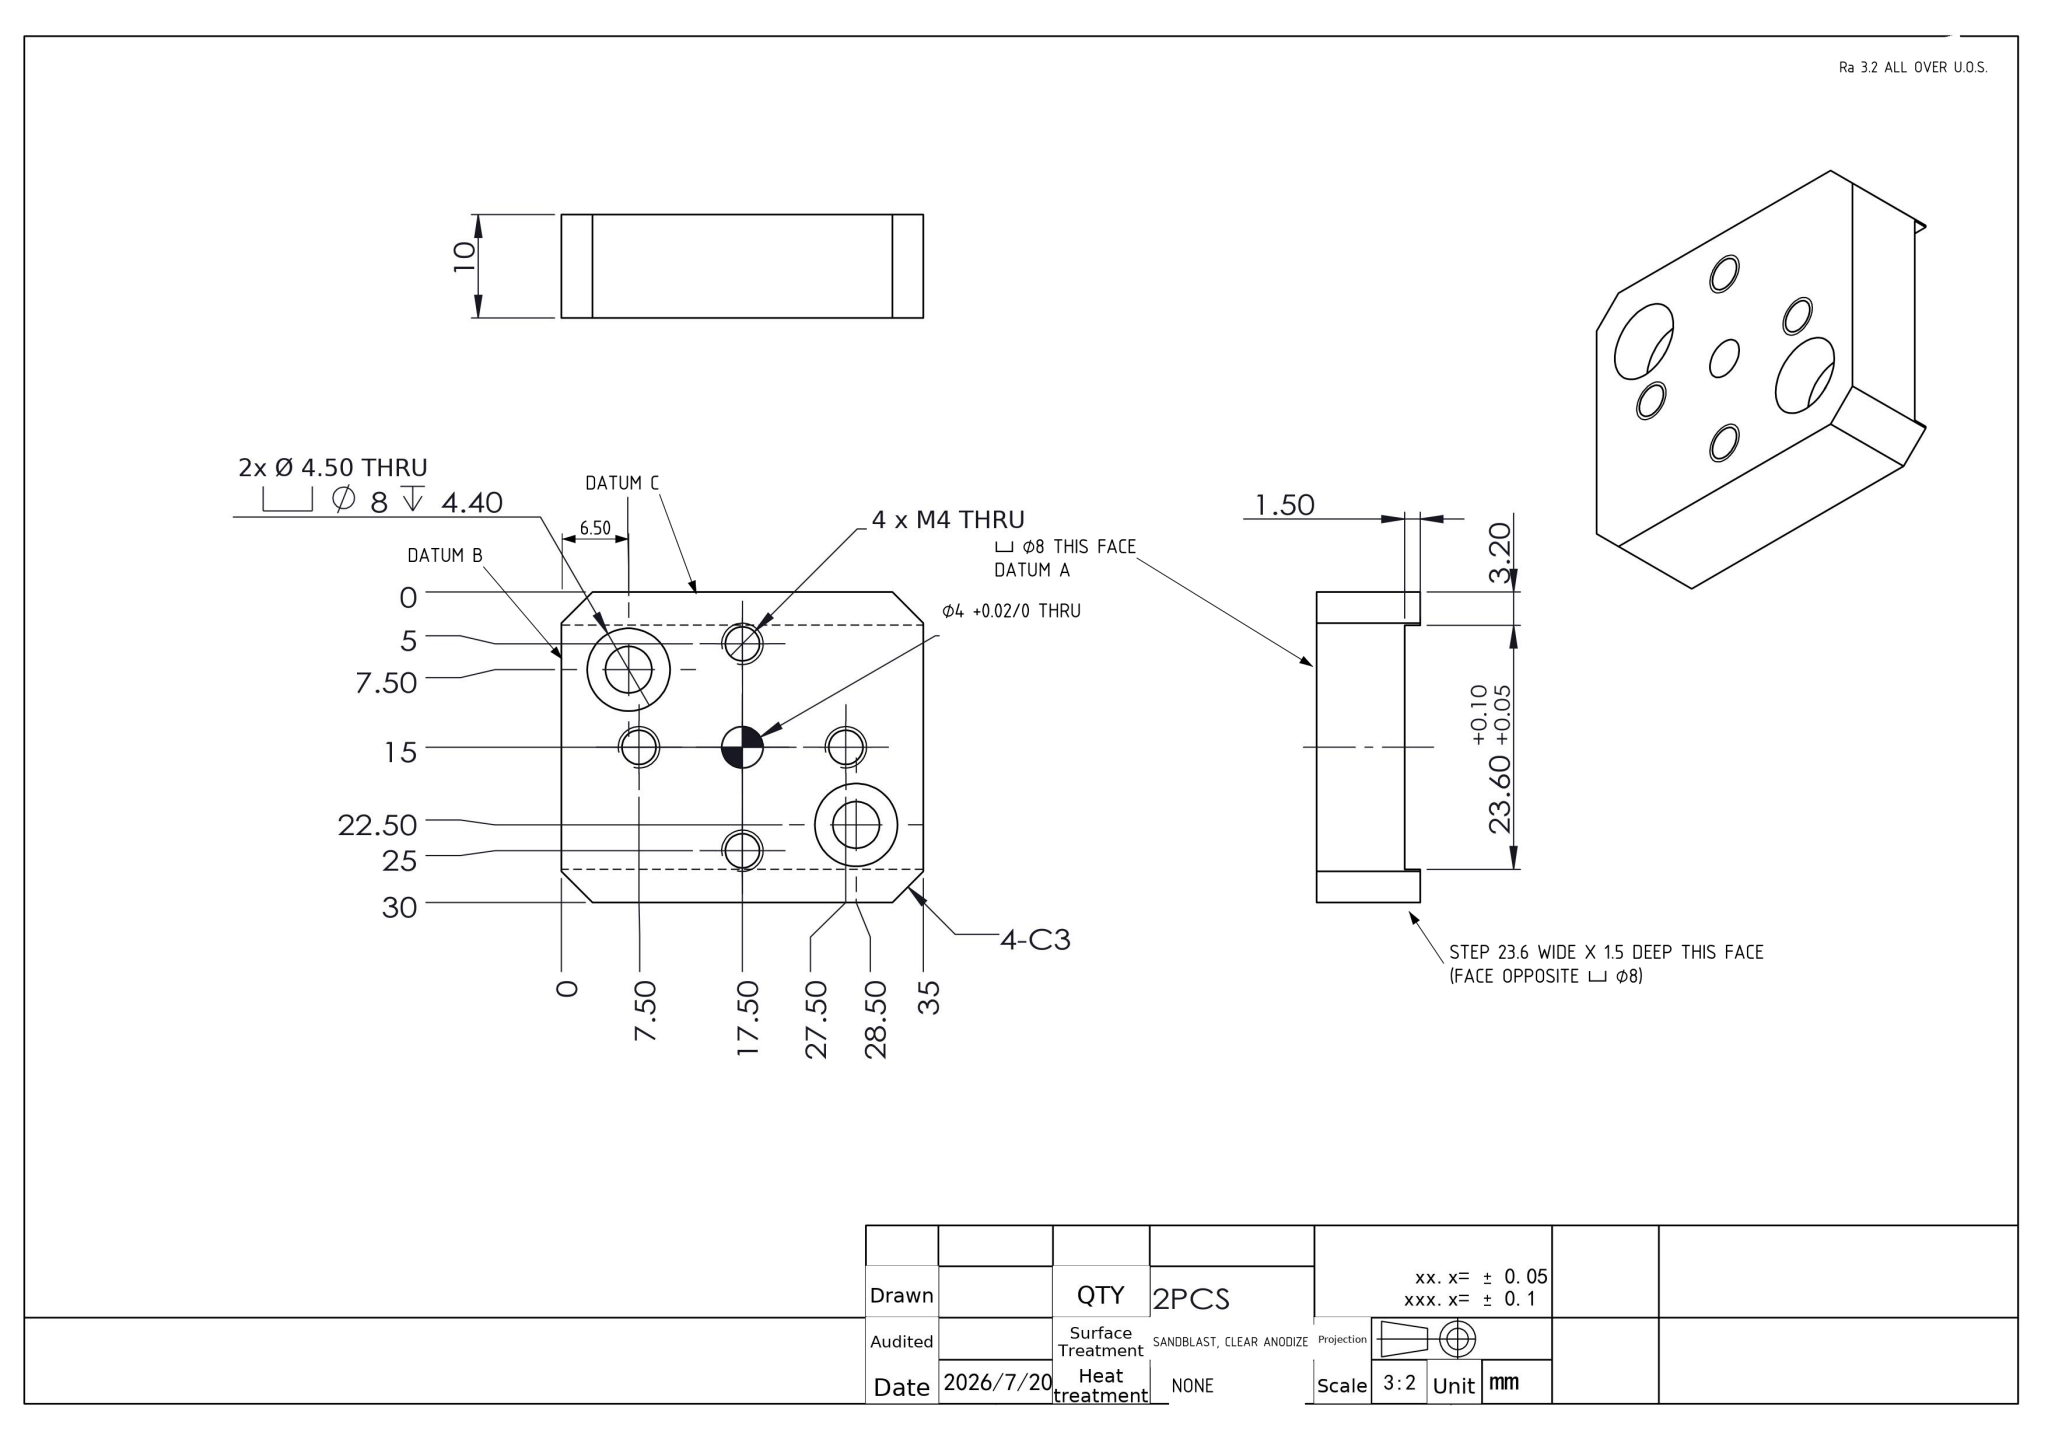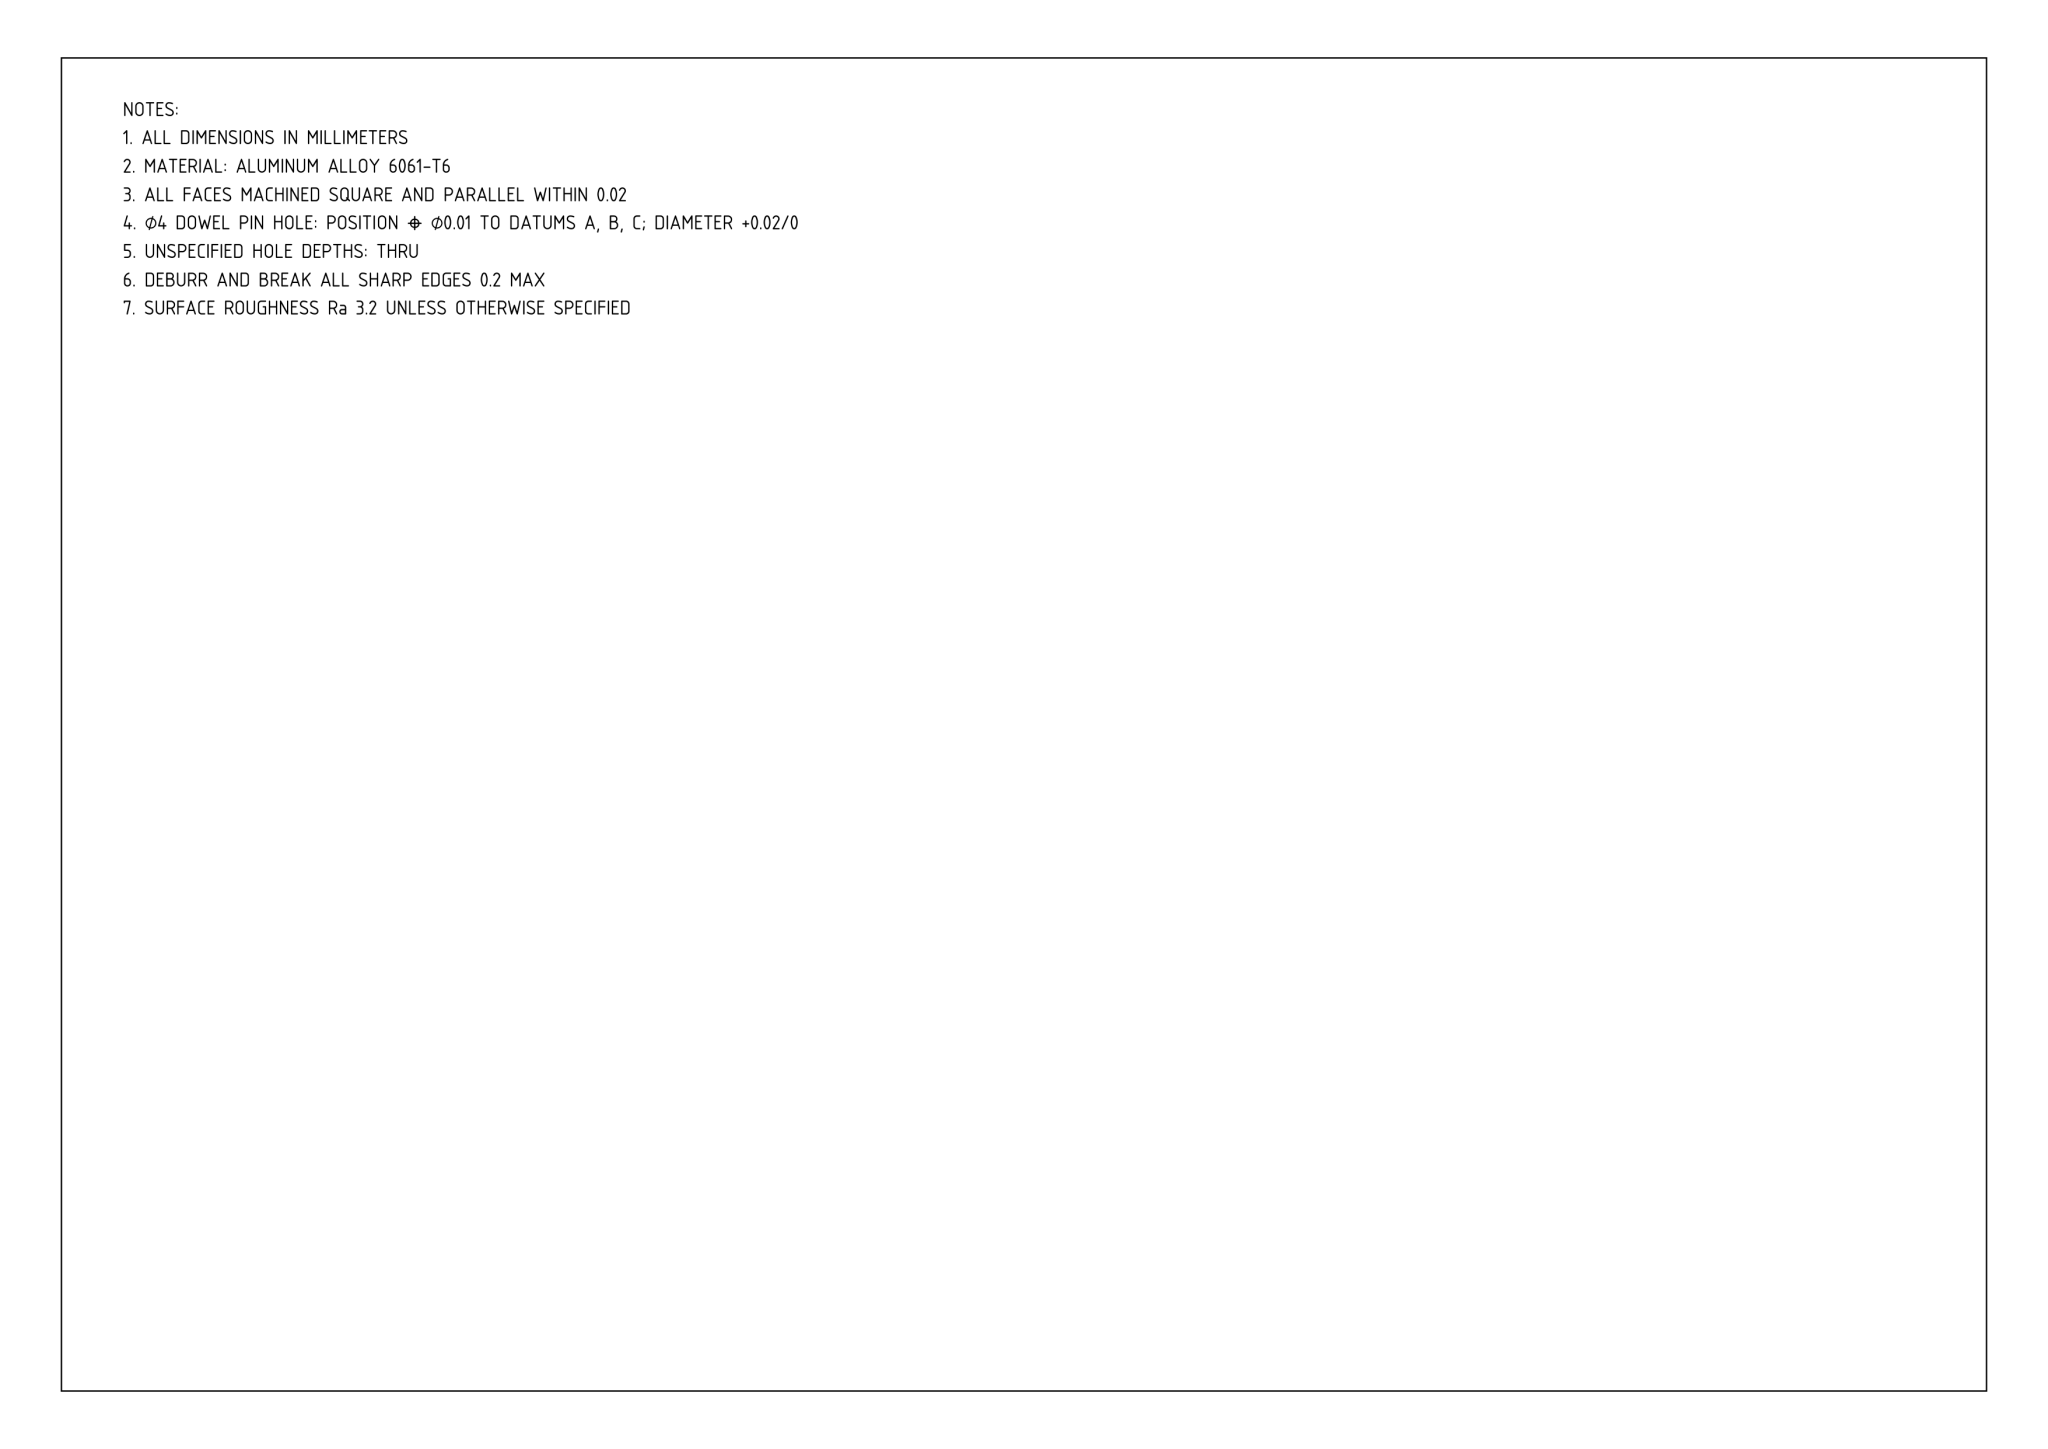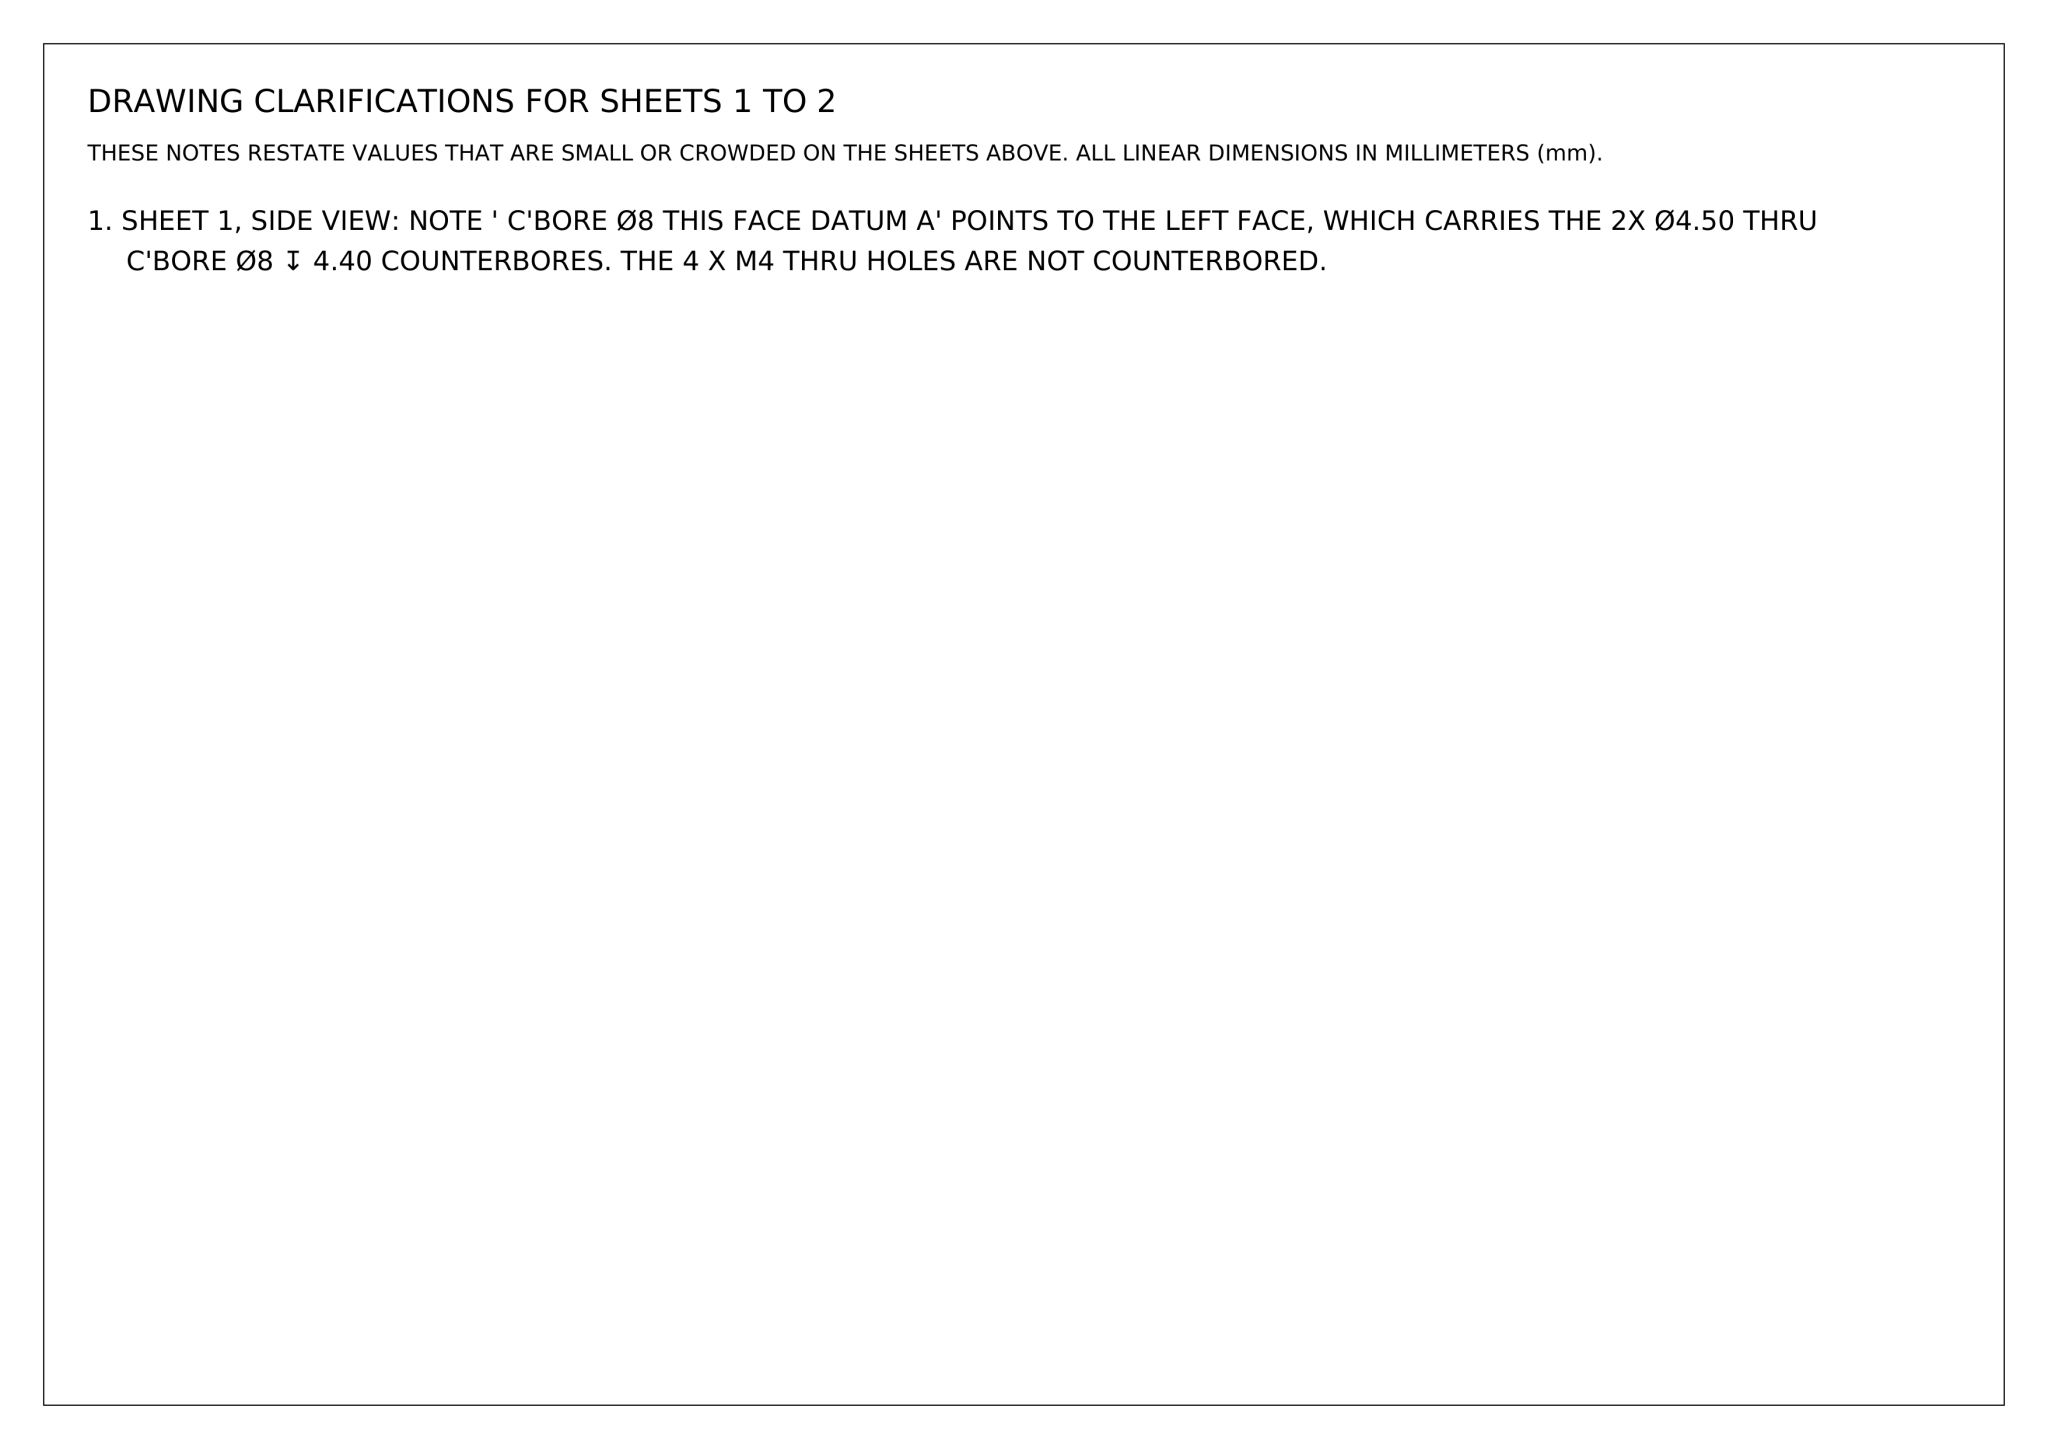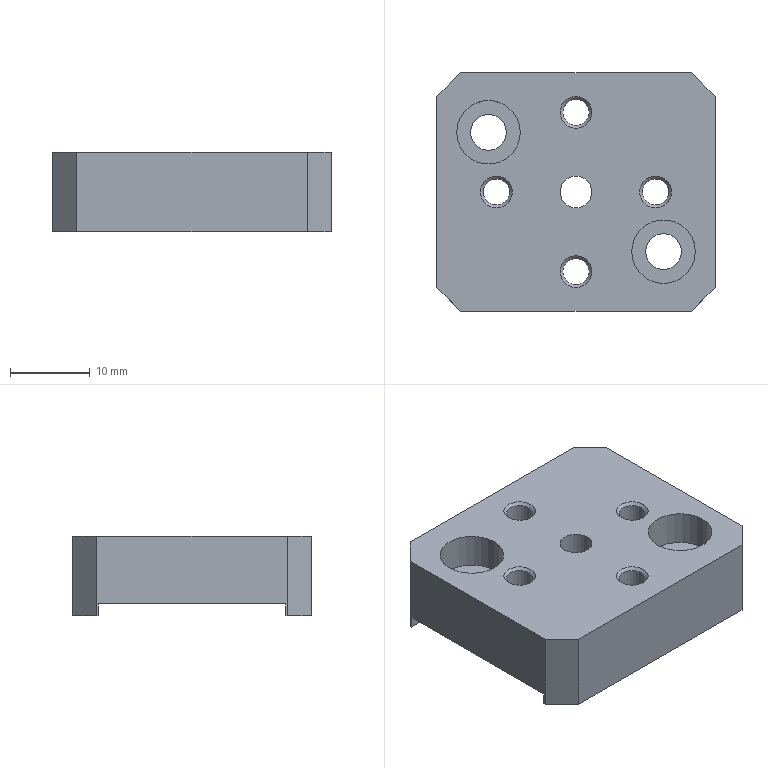Part | NX | mm | 1 solid | 31 faces | box 35 x 30 x 10 mm | volume 8108 mm3 | plane 16 | cylinder 9 | cone 6 | commonest cylinder face diameters 3.3 x4 4.5 x2 8 x2 4 x1